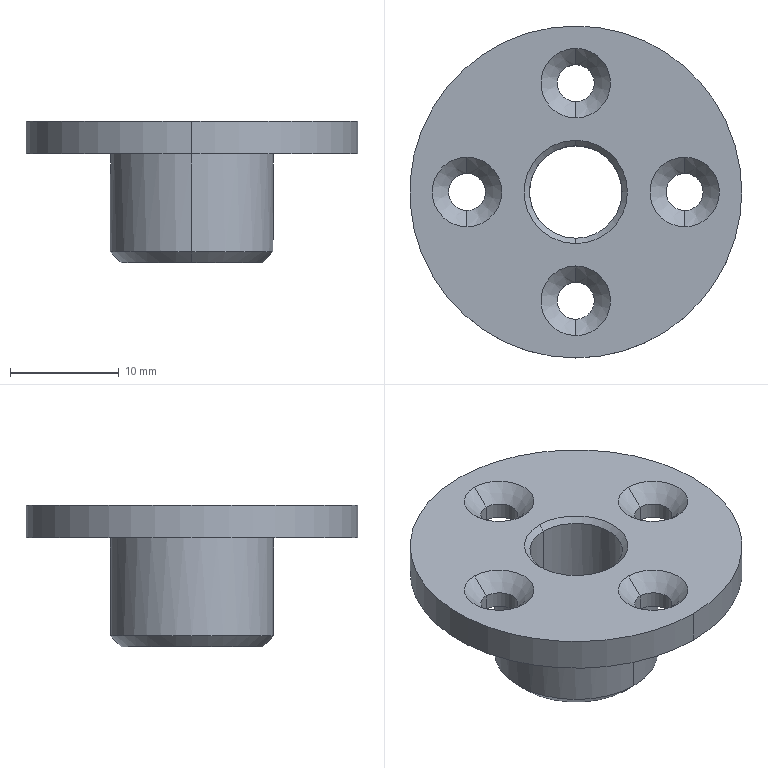CAM job | Mastercam | mm | 1 operations | part box 30.5 x 30.5 x 13
1. Drill/Counterbore | 7 - 4 倒角刀